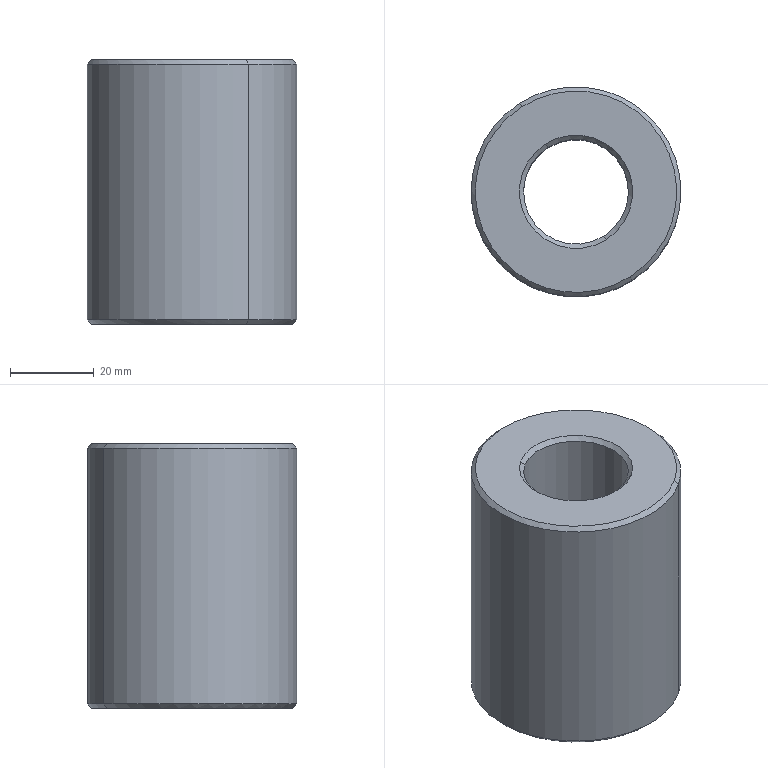Component | SolidWorks | GL-56x64-15-25LightCoupling-1 | 1 solid | 12 faces | box 50 x 50 x 63 mm | volume 92580 mm3 | cone 6 | cylinder 4 | plane 2 | commonest cylinder face diameters 25 x2 50 x2
build123d program:
from build123d import *

# Parameters (mm, degrees)
SKETCH1_R           = 25
BOSS_EXTRUDE1_DEPTH = 63
SKETCH2_R           = 12.5
CUT_EXTRUDE1_DEPTH  = 73.243
CHAMFER1_SIZE       = 1


with BuildPart() as part:
    # Sketch1 → Boss-Extrude1 (new body)
    with BuildSketch(Plane(origin=(0, 0, 0), x_dir=(1, 0, 0), z_dir=(0, 1, 0))):
        with Locations(Location((0, 0, 0), (0, 0, 270))):
            Circle(SKETCH1_R)
    extrude(amount=BOSS_EXTRUDE1_DEPTH)

    # Sketch2 → Cut-Extrude1 (cut, through all)
    with BuildSketch(Plane.XZ):
        with Locations(Location((0, 0, 0), (0, 0, 270))):
            Circle(SKETCH2_R)
    extrude(amount=-CUT_EXTRUDE1_DEPTH, mode=Mode.SUBTRACT)

    # Chamfer1
    chamfer1_edges = [part.edges().sort_by_distance(p)[0] for p in [
        (0, 0, -25),
        (0, 63, -25),
        (0, 63, 12.5),
    ]]
    chamfer(chamfer1_edges, length=CHAMFER1_SIZE)


solid = part.part

# Placed as in the assembly
solid = solid.moved(Location((733.029, 200.722, -81.5), (90, 0, 0)))
STEP:
#1=COLOUR_RGB('',0.7922,0.8196,0.9333);
#2=FILL_AREA_STYLE_COLOUR('',#1);
#3=FILL_AREA_STYLE('',(#2));
#4=SURFACE_STYLE_FILL_AREA(#3);
#5=SURFACE_SIDE_STYLE('',(#4));
#6=SURFACE_STYLE_USAGE(.BOTH.,#5);
#7=PRESENTATION_STYLE_ASSIGNMENT((#6));
#8=CARTESIAN_POINT('',(28.351,8.699,-3.209));
#9=VERTEX_POINT('',#8);
#10=CARTESIAN_POINT('',(29.368,7.106,-3.209));
#11=VERTEX_POINT('',#10);
#12=CARTESIAN_POINT('',(28.859,7.902,-3.209));
#13=DIRECTION('',(-0.,-0.,-1.));
#14=DIRECTION('',(0.538,-0.8429,0.));
#15=AXIS2_PLACEMENT_3D('',#12,#13,#14);
#16=CIRCLE('',#15,0.9449);
#17=EDGE_CURVE('',#9,#11,#16,.T.);
#18=ORIENTED_EDGE('',*,*,#17,.F.);
#19=CARTESIAN_POINT('',(28.33,8.732,-3.169));
#20=VERTEX_POINT('',#19);
#21=CARTESIAN_POINT('',(28.33,8.732,-3.169));
#22=DIRECTION('',(-0.3804,0.596,0.7071));
#23=VECTOR('',#22,39.37);
#24=LINE('',#21,#23);
#25=EDGE_CURVE('',#9,#20,#24,.T.);
#26=ORIENTED_EDGE('',*,*,#25,.T.);
#27=CARTESIAN_POINT('',(29.389,7.073,-3.169));
#28=VERTEX_POINT('',#27);
#29=CARTESIAN_POINT('',(28.859,7.902,-3.169));
#30=DIRECTION('',(0.,0.,1.));
#31=DIRECTION('',(0.538,-0.8429,0.));
#32=AXIS2_PLACEMENT_3D('',#29,#30,#31);
#33=CIRCLE('',#32,0.9843);
#34=EDGE_CURVE('',#28,#20,#33,.T.);
#35=ORIENTED_EDGE('',*,*,#34,.F.);
#36=CARTESIAN_POINT('',(29.389,7.073,-3.169));
#37=DIRECTION('',(0.3804,-0.596,0.7071));
#38=VECTOR('',#37,39.37);
#39=LINE('',#36,#38);
#40=EDGE_CURVE('',#11,#28,#39,.T.);
#41=ORIENTED_EDGE('',*,*,#40,.F.);
#42=EDGE_LOOP('',(#18,#26,#35,#41));
#43=FACE_OUTER_BOUND('',#42,.T.);
#44=CARTESIAN_POINT('',(28.859,7.902,-3.169));
#45=DIRECTION('',(0.,0.,1.));
#46=DIRECTION('',(0.538,-0.8429,0.));
#47=AXIS2_PLACEMENT_3D('',#44,#45,#46);
#48=CONICAL_SURFACE('',#47,0.9843,0.7854);
#49=ADVANCED_FACE('',(#43),#48,.T.);
#50=CARTESIAN_POINT('',(28.595,8.317,-0.7677));
#51=VERTEX_POINT('',#50);
#52=CARTESIAN_POINT('',(29.124,7.488,-0.7677));
#53=VERTEX_POINT('',#52);
#54=CARTESIAN_POINT('',(28.859,7.902,-0.7677));
#55=DIRECTION('',(0.,0.,1.));
#56=DIRECTION('',(0.538,-0.8429,0.));
#57=AXIS2_PLACEMENT_3D('',#54,#55,#56);
#58=CIRCLE('',#57,0.4921);
#59=EDGE_CURVE('',#51,#53,#58,.T.);
#60=ORIENTED_EDGE('',*,*,#59,.F.);
#61=CARTESIAN_POINT('',(28.573,8.35,-0.7283));
#62=VERTEX_POINT('',#61);
#63=CARTESIAN_POINT('',(28.573,8.35,-0.7283));
#64=DIRECTION('',(-0.3804,0.596,0.7071));
#65=VECTOR('',#64,39.37);
#66=LINE('',#63,#65);
#67=EDGE_CURVE('',#51,#62,#66,.T.);
#68=ORIENTED_EDGE('',*,*,#67,.T.);
#69=CARTESIAN_POINT('',(29.145,7.454,-0.7283));
#70=VERTEX_POINT('',#69);
#71=CARTESIAN_POINT('',(28.859,7.902,-0.7283));
#72=DIRECTION('',(-0.,-0.,-1.));
#73=DIRECTION('',(0.538,-0.8429,0.));
#74=AXIS2_PLACEMENT_3D('',#71,#72,#73);
#75=CIRCLE('',#74,0.5315);
#76=EDGE_CURVE('',#70,#62,#75,.T.);
#77=ORIENTED_EDGE('',*,*,#76,.F.);
#78=CARTESIAN_POINT('',(29.145,7.454,-0.7283));
#79=DIRECTION('',(0.3804,-0.596,0.7071));
#80=VECTOR('',#79,39.37);
#81=LINE('',#78,#80);
#82=EDGE_CURVE('',#53,#70,#81,.T.);
#83=ORIENTED_EDGE('',*,*,#82,.F.);
#84=EDGE_LOOP('',(#60,#68,#77,#83));
#85=FACE_OUTER_BOUND('',#84,.T.);
#86=CARTESIAN_POINT('',(28.859,7.902,-0.7283));
#87=DIRECTION('',(0.,0.,1.));
#88=DIRECTION('',(0.538,-0.8429,0.));
#89=AXIS2_PLACEMENT_3D('',#86,#87,#88);
#90=CONICAL_SURFACE('',#89,0.5315,0.7854);
#91=ADVANCED_FACE('',(#85),#90,.F.);
#92=CARTESIAN_POINT('',(29.368,7.106,-0.7283));
#93=VERTEX_POINT('',#92);
#94=CARTESIAN_POINT('',(28.351,8.699,-0.7283));
#95=VERTEX_POINT('',#94);
#96=CARTESIAN_POINT('',(28.859,7.902,-0.7283));
#97=DIRECTION('',(0.,0.,1.));
#98=DIRECTION('',(0.538,-0.8429,0.));
#99=AXIS2_PLACEMENT_3D('',#96,#97,#98);
#100=CIRCLE('',#99,0.9449);
#101=EDGE_CURVE('',#93,#95,#100,.T.);
#102=ORIENTED_EDGE('',*,*,#101,.F.);
#103=CARTESIAN_POINT('',(29.389,7.073,-0.7677));
#104=VERTEX_POINT('',#103);
#105=CARTESIAN_POINT('',(29.368,7.106,-0.7283));
#106=DIRECTION('',(0.3804,-0.596,-0.7071));
#107=VECTOR('',#106,39.37);
#108=LINE('',#105,#107);
#109=EDGE_CURVE('',#93,#104,#108,.T.);
#110=ORIENTED_EDGE('',*,*,#109,.T.);
#111=CARTESIAN_POINT('',(28.33,8.732,-0.7677));
#112=VERTEX_POINT('',#111);
#113=CARTESIAN_POINT('',(28.859,7.902,-0.7677));
#114=DIRECTION('',(-0.,-0.,-1.));
#115=DIRECTION('',(0.538,-0.8429,0.));
#116=AXIS2_PLACEMENT_3D('',#113,#114,#115);
#117=CIRCLE('',#116,0.9843);
#118=EDGE_CURVE('',#112,#104,#117,.T.);
#119=ORIENTED_EDGE('',*,*,#118,.F.);
#120=CARTESIAN_POINT('',(28.351,8.699,-0.7283));
#121=DIRECTION('',(-0.3804,0.596,-0.7071));
#122=VECTOR('',#121,39.37);
#123=LINE('',#120,#122);
#124=EDGE_CURVE('',#95,#112,#123,.T.);
#125=ORIENTED_EDGE('',*,*,#124,.F.);
#126=EDGE_LOOP('',(#102,#110,#119,#125));
#127=FACE_OUTER_BOUND('',#126,.T.);
#128=CARTESIAN_POINT('',(28.859,7.902,-0.7283));
#129=DIRECTION('',(-0.,-0.,-1.));
#130=DIRECTION('',(-0.538,0.8429,0.));
#131=AXIS2_PLACEMENT_3D('',#128,#129,#130);
#132=CONICAL_SURFACE('',#131,0.9449,0.7854);
#133=ADVANCED_FACE('',(#127),#132,.T.);
#134=ORIENTED_EDGE('',*,*,#59,.T.);
#135=CARTESIAN_POINT('',(29.124,7.488,-3.209));
#136=VERTEX_POINT('',#135);
#137=CARTESIAN_POINT('',(29.124,7.488,-0.7283));
#138=DIRECTION('',(-0.,-0.,-1.));
#139=VECTOR('',#138,39.37);
#140=LINE('',#137,#139);
#141=EDGE_CURVE('',#53,#136,#140,.T.);
#142=ORIENTED_EDGE('',*,*,#141,.T.);
#143=CARTESIAN_POINT('',(28.595,8.317,-3.209));
#144=VERTEX_POINT('',#143);
#145=CARTESIAN_POINT('',(28.859,7.902,-3.209));
#146=DIRECTION('',(-0.,-0.,-1.));
#147=DIRECTION('',(-0.538,0.8429,0.));
#148=AXIS2_PLACEMENT_3D('',#145,#146,#147);
#149=CIRCLE('',#148,0.4921);
#150=EDGE_CURVE('',#136,#144,#149,.T.);
#151=ORIENTED_EDGE('',*,*,#150,.T.);
#152=CARTESIAN_POINT('',(28.595,8.317,-0.7283));
#153=DIRECTION('',(-0.,-0.,-1.));
#154=VECTOR('',#153,39.37);
#155=LINE('',#152,#154);
#156=EDGE_CURVE('',#51,#144,#155,.T.);
#157=ORIENTED_EDGE('',*,*,#156,.F.);
#158=EDGE_LOOP('',(#134,#142,#151,#157));
#159=FACE_OUTER_BOUND('',#158,.T.);
#160=CARTESIAN_POINT('',(28.859,7.902,-0.7283));
#161=DIRECTION('',(-0.,-0.,-1.));
#162=DIRECTION('',(-0.538,0.8429,0.));
#163=AXIS2_PLACEMENT_3D('',#160,#161,#162);
#164=CYLINDRICAL_SURFACE('',#163,0.4921);
#165=ADVANCED_FACE('',(#159),#164,.F.);
#166=ORIENTED_EDGE('',*,*,#118,.T.);
#167=CARTESIAN_POINT('',(29.389,7.073,-0.7283));
#168=DIRECTION('',(-0.,-0.,-1.));
#169=VECTOR('',#168,39.37);
#170=LINE('',#167,#169);
#171=EDGE_CURVE('',#104,#28,#170,.T.);
#172=ORIENTED_EDGE('',*,*,#171,.T.);
#173=ORIENTED_EDGE('',*,*,#34,.T.);
#174=CARTESIAN_POINT('',(28.33,8.732,-0.7283));
#175=DIRECTION('',(-0.,-0.,-1.));
#176=VECTOR('',#175,39.37);
#177=LINE('',#174,#176);
#178=EDGE_CURVE('',#112,#20,#177,.T.);
#179=ORIENTED_EDGE('',*,*,#178,.F.);
#180=EDGE_LOOP('',(#166,#172,#173,#179));
#181=FACE_OUTER_BOUND('',#180,.T.);
#182=CARTESIAN_POINT('',(28.859,7.902,-0.7283));
#183=DIRECTION('',(-0.,-0.,-1.));
#184=DIRECTION('',(-0.538,0.8429,0.));
#185=AXIS2_PLACEMENT_3D('',#182,#183,#184);
#186=CYLINDRICAL_SURFACE('',#185,0.9843);
#187=ADVANCED_FACE('',(#181),#186,.T.);
#188=ORIENTED_EDGE('',*,*,#171,.F.);
#189=CARTESIAN_POINT('',(28.859,7.902,-0.7677));
#190=DIRECTION('',(-0.,-0.,-1.));
#191=DIRECTION('',(0.538,-0.8429,0.));
#192=AXIS2_PLACEMENT_3D('',#189,#190,#191);
#193=CIRCLE('',#192,0.9843);
#194=EDGE_CURVE('',#104,#112,#193,.T.);
#195=ORIENTED_EDGE('',*,*,#194,.T.);
#196=ORIENTED_EDGE('',*,*,#178,.T.);
#197=CARTESIAN_POINT('',(28.859,7.902,-3.169));
#198=DIRECTION('',(0.,0.,1.));
#199=DIRECTION('',(0.538,-0.8429,0.));
#200=AXIS2_PLACEMENT_3D('',#197,#198,#199);
#201=CIRCLE('',#200,0.9843);
#202=EDGE_CURVE('',#20,#28,#201,.T.);
#203=ORIENTED_EDGE('',*,*,#202,.T.);
#204=EDGE_LOOP('',(#188,#195,#196,#203));
#205=FACE_OUTER_BOUND('',#204,.T.);
#206=CARTESIAN_POINT('',(28.859,7.902,-0.7283));
#207=DIRECTION('',(-0.,-0.,-1.));
#208=DIRECTION('',(-0.538,0.8429,0.));
#209=AXIS2_PLACEMENT_3D('',#206,#207,#208);
#210=CYLINDRICAL_SURFACE('',#209,0.9843);
#211=ADVANCED_FACE('',(#205),#210,.T.);
#212=CARTESIAN_POINT('',(28.859,7.902,-0.7283));
#213=DIRECTION('',(0.,0.,1.));
#214=DIRECTION('',(0.538,-0.8429,0.));
#215=AXIS2_PLACEMENT_3D('',#212,#213,#214);
#216=CIRCLE('',#215,0.9449);
#217=EDGE_CURVE('',#95,#93,#216,.T.);
#218=ORIENTED_EDGE('',*,*,#217,.T.);
#219=ORIENTED_EDGE('',*,*,#101,.T.);
#220=EDGE_LOOP('',(#218,#219));
#221=FACE_OUTER_BOUND('',#220,.T.);
#222=ORIENTED_EDGE('',*,*,#76,.T.);
#223=CARTESIAN_POINT('',(28.859,7.902,-0.7283));
#224=DIRECTION('',(-0.,-0.,-1.));
#225=DIRECTION('',(0.538,-0.8429,0.));
#226=AXIS2_PLACEMENT_3D('',#223,#224,#225);
#227=CIRCLE('',#226,0.5315);
#228=EDGE_CURVE('',#62,#70,#227,.T.);
#229=ORIENTED_EDGE('',*,*,#228,.T.);
#230=EDGE_LOOP('',(#222,#229));
#231=FACE_BOUND('',#230,.T.);
#232=CARTESIAN_POINT('',(28.859,7.902,-0.7283));
#233=DIRECTION('',(0.,0.,1.));
#234=DIRECTION('',(0.538,-0.8429,0.));
#235=AXIS2_PLACEMENT_3D('',#232,#233,#234);
#236=PLANE('',#235);
#237=ADVANCED_FACE('',(#221,#231),#236,.T.);
#238=CARTESIAN_POINT('',(28.859,7.902,-3.209));
#239=DIRECTION('',(-0.,-0.,-1.));
#240=DIRECTION('',(0.538,-0.8429,0.));
#241=AXIS2_PLACEMENT_3D('',#238,#239,#240);
#242=CIRCLE('',#241,0.9449);
#243=EDGE_CURVE('',#11,#9,#242,.T.);
#244=ORIENTED_EDGE('',*,*,#243,.T.);
#245=ORIENTED_EDGE('',*,*,#17,.T.);
#246=EDGE_LOOP('',(#244,#245));
#247=FACE_OUTER_BOUND('',#246,.T.);
#248=CARTESIAN_POINT('',(28.859,7.902,-3.209));
#249=DIRECTION('',(-0.,-0.,-1.));
#250=DIRECTION('',(-0.538,0.8429,0.));
#251=AXIS2_PLACEMENT_3D('',#248,#249,#250);
#252=CIRCLE('',#251,0.4921);
#253=EDGE_CURVE('',#144,#136,#252,.T.);
#254=ORIENTED_EDGE('',*,*,#253,.F.);
#255=ORIENTED_EDGE('',*,*,#150,.F.);
#256=EDGE_LOOP('',(#254,#255));
#257=FACE_BOUND('',#256,.T.);
#258=CARTESIAN_POINT('',(28.859,7.902,-3.209));
#259=DIRECTION('',(0.,0.,1.));
#260=DIRECTION('',(0.538,-0.8429,0.));
#261=AXIS2_PLACEMENT_3D('',#258,#259,#260);
#262=PLANE('',#261);
#263=ADVANCED_FACE('',(#247,#257),#262,.F.);
#264=ORIENTED_EDGE('',*,*,#141,.F.);
#265=CARTESIAN_POINT('',(28.859,7.902,-0.7677));
#266=DIRECTION('',(0.,0.,1.));
#267=DIRECTION('',(0.538,-0.8429,0.));
#268=AXIS2_PLACEMENT_3D('',#265,#266,#267);
#269=CIRCLE('',#268,0.4921);
#270=EDGE_CURVE('',#53,#51,#269,.T.);
#271=ORIENTED_EDGE('',*,*,#270,.T.);
#272=ORIENTED_EDGE('',*,*,#156,.T.);
#273=ORIENTED_EDGE('',*,*,#253,.T.);
#274=EDGE_LOOP('',(#264,#271,#272,#273));
#275=FACE_OUTER_BOUND('',#274,.T.);
#276=CARTESIAN_POINT('',(28.859,7.902,-0.7283));
#277=DIRECTION('',(-0.,-0.,-1.));
#278=DIRECTION('',(-0.538,0.8429,0.));
#279=AXIS2_PLACEMENT_3D('',#276,#277,#278);
#280=CYLINDRICAL_SURFACE('',#279,0.4921);
#281=ADVANCED_FACE('',(#275),#280,.F.);
#282=ORIENTED_EDGE('',*,*,#109,.F.);
#283=ORIENTED_EDGE('',*,*,#217,.F.);
#284=ORIENTED_EDGE('',*,*,#124,.T.);
#285=ORIENTED_EDGE('',*,*,#194,.F.);
#286=EDGE_LOOP('',(#282,#283,#284,#285));
#287=FACE_OUTER_BOUND('',#286,.T.);
#288=CARTESIAN_POINT('',(28.859,7.902,-0.7283));
#289=DIRECTION('',(-0.,-0.,-1.));
#290=DIRECTION('',(-0.538,0.8429,0.));
#291=AXIS2_PLACEMENT_3D('',#288,#289,#290);
#292=CONICAL_SURFACE('',#291,0.9449,0.7854);
#293=ADVANCED_FACE('',(#287),#292,.T.);
#294=ORIENTED_EDGE('',*,*,#67,.F.);
#295=ORIENTED_EDGE('',*,*,#270,.F.);
#296=ORIENTED_EDGE('',*,*,#82,.T.);
#297=ORIENTED_EDGE('',*,*,#228,.F.);
#298=EDGE_LOOP('',(#294,#295,#296,#297));
#299=FACE_OUTER_BOUND('',#298,.T.);
#300=CARTESIAN_POINT('',(28.859,7.902,-0.7283));
#301=DIRECTION('',(0.,0.,1.));
#302=DIRECTION('',(0.538,-0.8429,0.));
#303=AXIS2_PLACEMENT_3D('',#300,#301,#302);
#304=CONICAL_SURFACE('',#303,0.5315,0.7854);
#305=ADVANCED_FACE('',(#299),#304,.F.);
#306=ORIENTED_EDGE('',*,*,#25,.F.);
#307=ORIENTED_EDGE('',*,*,#243,.F.);
#308=ORIENTED_EDGE('',*,*,#40,.T.);
#309=ORIENTED_EDGE('',*,*,#202,.F.);
#310=EDGE_LOOP('',(#306,#307,#308,#309));
#311=FACE_OUTER_BOUND('',#310,.T.);
#312=CARTESIAN_POINT('',(28.859,7.902,-3.169));
#313=DIRECTION('',(0.,0.,1.));
#314=DIRECTION('',(0.538,-0.8429,0.));
#315=AXIS2_PLACEMENT_3D('',#312,#313,#314);
#316=CONICAL_SURFACE('',#315,0.9843,0.7854);
#317=ADVANCED_FACE('',(#311),#316,.T.);
#318=CLOSED_SHELL('',(#49,#91,#133,#165,#187,#211,#237,#263,#281,#293,#305,#317));
#319=MANIFOLD_SOLID_BREP('',#318);
#320=STYLED_ITEM('',(#7),#319);
#321=PRESENTATION_LAYER_ASSIGNMENT('','',(#320));
#322=CARTESIAN_POINT('',(0.,0.,0.));
#323=DIRECTION('',(0.,0.,1.));
#324=DIRECTION('',(1.,0.,0.));
#325=AXIS2_PLACEMENT_3D('',#322,#323,#324);
#326=(LENGTH_UNIT()NAMED_UNIT(*)SI_UNIT($,.METRE.));
#327=LENGTH_MEASURE_WITH_UNIT(LENGTH_MEASURE(0.0254),#326);
#328=DIMENSIONAL_EXPONENTS(1.,0.,0.,0.,0.,0.,0.);
#329=(CONVERSION_BASED_UNIT('',#327)LENGTH_UNIT()NAMED_UNIT(#328));
#330=UNCERTAINTY_MEASURE_WITH_UNIT(LENGTH_MEASURE(0.00001),#329,'','');
#331=(NAMED_UNIT(*)PLANE_ANGLE_UNIT()SI_UNIT($,.RADIAN.));
#332=(NAMED_UNIT(*)SI_UNIT($,.STERADIAN.)SOLID_ANGLE_UNIT());
#333=(GEOMETRIC_REPRESENTATION_CONTEXT(3)GLOBAL_UNCERTAINTY_ASSIGNED_CONTEXT((#330))GLOBAL_UNIT_ASSIGNED_CONTEXT((#329,#331,#332))REPRESENTATION_CONTEXT('',''));
#334=ADVANCED_BREP_SHAPE_REPRESENTATION('',(#319,#325),#333);
#335=(LENGTH_UNIT()NAMED_UNIT(*)SI_UNIT($,.METRE.));
#336=LENGTH_MEASURE_WITH_UNIT(LENGTH_MEASURE(0.0254),#335);
#337=DIMENSIONAL_EXPONENTS(1.,0.,0.,0.,0.,0.,0.);
#338=(CONVERSION_BASED_UNIT('',#336)LENGTH_UNIT()NAMED_UNIT(#337));
#339=UNCERTAINTY_MEASURE_WITH_UNIT(LENGTH_MEASURE(0.00001),#338,'','');
#340=(NAMED_UNIT(*)PLANE_ANGLE_UNIT()SI_UNIT($,.RADIAN.));
#341=(NAMED_UNIT(*)SI_UNIT($,.STERADIAN.)SOLID_ANGLE_UNIT());
#342=(GEOMETRIC_REPRESENTATION_CONTEXT(3)GLOBAL_UNCERTAINTY_ASSIGNED_CONTEXT((#339))GLOBAL_UNIT_ASSIGNED_CONTEXT((#338,#340,#341))REPRESENTATION_CONTEXT('',''));
#343=MECHANICAL_DESIGN_GEOMETRIC_PRESENTATION_REPRESENTATION('',(#320),#342);